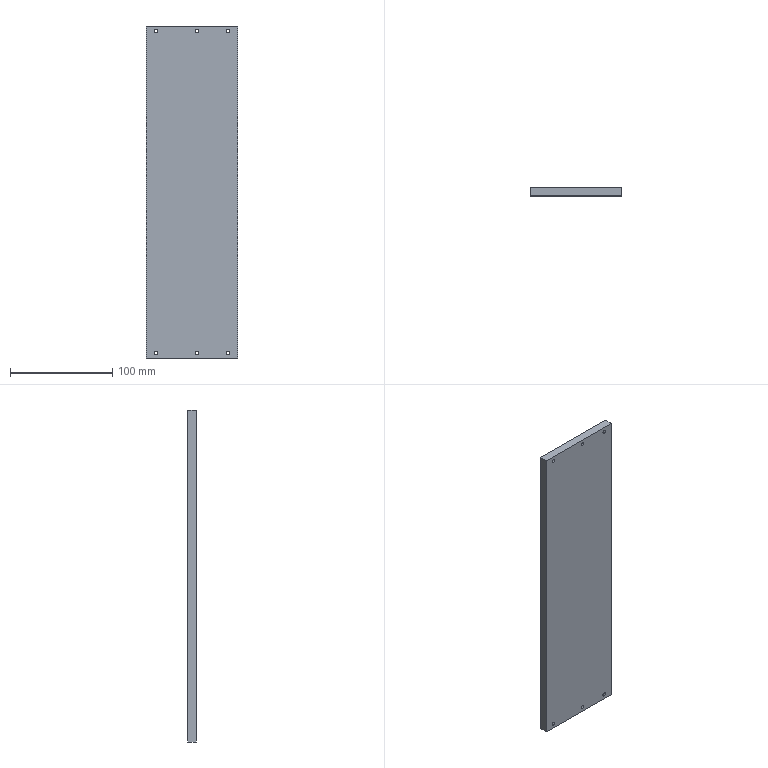Component | SolidWorks | Q1-A12-S21-Q4-12A-1 | 1 solid | 36 faces | box 90 x 8 x 325 mm | volume 233130 mm3 | cylinder 24 | plane 12 | commonest cylinder face diameters 6.5 x12 3.4 x12 | material White Plastic Steel POM
build123d program:
from build123d import *

# Parameters (mm, degrees)
SKETCH1_W                                            = 325
SKETCH1_H                                            = 90
BOSS_EXTRUDE1_DEPTH                                  = 8
M3_SOCKET_HEAD_CAP_SCREW_CYLINDRICAL_COU_D           = 3.4
M3_SOCKET_HEAD_CAP_SCREW_CYLINDRICAL_COU_CBORE_D     = 6.5
M3_SOCKET_HEAD_CAP_SCREW_CYLINDRICAL_COU_CBORE_DEPTH = 3


with BuildPart() as part:
    # Sketch1 → Boss-Extrude1 (new body)
    with BuildSketch(Plane(origin=(0, 0, 0), x_dir=(1, 0, 0), z_dir=(0, 1, 0))):
        Rectangle(SKETCH1_W, SKETCH1_H)
    extrude(amount=BOSS_EXTRUDE1_DEPTH)

    # M3 Socket Head Cap Screw Cylindrical Cou (through all)
    with Locations(Plane(origin=(0, 8, 0), x_dir=(1, 0, 0), z_dir=(0, 1, 0))):
        with Locations((157.5, 35), (157.5, 5), (157.5, -35), (-157.5, 35), (-157.5, 5), (-157.5, -35)):
            CounterBoreHole(M3_SOCKET_HEAD_CAP_SCREW_CYLINDRICAL_COU_D / 2, M3_SOCKET_HEAD_CAP_SCREW_CYLINDRICAL_COU_CBORE_D / 2, M3_SOCKET_HEAD_CAP_SCREW_CYLINDRICAL_COU_CBORE_DEPTH)


solid = part.part

# Placed as in the assembly
solid = solid.moved(Location((263.5, 180, 0), (0, -90, 0)))
STEP:
#1=COLOUR_RGB('',0.7922,0.8196,0.9333);
#2=FILL_AREA_STYLE_COLOUR('',#1);
#3=FILL_AREA_STYLE('',(#2));
#4=SURFACE_STYLE_FILL_AREA(#3);
#5=SURFACE_SIDE_STYLE('',(#4));
#6=SURFACE_STYLE_USAGE(.BOTH.,#5);
#7=PRESENTATION_STYLE_ASSIGNMENT((#6));
#8=CARTESIAN_POINT('',(11.88,7.283,6.201));
#9=VERTEX_POINT('',#8);
#10=CARTESIAN_POINT('',(11.624,7.283,6.201));
#11=VERTEX_POINT('',#10);
#12=CARTESIAN_POINT('',(11.752,7.283,6.201));
#13=DIRECTION('',(-0.,1.,0.));
#14=DIRECTION('',(-1.,0.,0.));
#15=AXIS2_PLACEMENT_3D('',#12,#13,#14);
#16=CIRCLE('',#15,0.128);
#17=EDGE_CURVE('',#9,#11,#16,.T.);
#18=ORIENTED_EDGE('',*,*,#17,.F.);
#19=CARTESIAN_POINT('',(11.88,7.402,6.201));
#20=VERTEX_POINT('',#19);
#21=CARTESIAN_POINT('',(11.88,7.402,6.201));
#22=DIRECTION('',(-0.,1.,0.));
#23=VECTOR('',#22,39.37);
#24=LINE('',#21,#23);
#25=EDGE_CURVE('',#9,#20,#24,.T.);
#26=ORIENTED_EDGE('',*,*,#25,.T.);
#27=CARTESIAN_POINT('',(11.624,7.402,6.201));
#28=VERTEX_POINT('',#27);
#29=CARTESIAN_POINT('',(11.752,7.402,6.201));
#30=DIRECTION('',(-0.,1.,0.));
#31=DIRECTION('',(-1.,0.,0.));
#32=AXIS2_PLACEMENT_3D('',#29,#30,#31);
#33=CIRCLE('',#32,0.128);
#34=EDGE_CURVE('',#20,#28,#33,.T.);
#35=ORIENTED_EDGE('',*,*,#34,.T.);
#36=CARTESIAN_POINT('',(11.624,7.402,6.201));
#37=DIRECTION('',(-0.,1.,0.));
#38=VECTOR('',#37,39.37);
#39=LINE('',#36,#38);
#40=EDGE_CURVE('',#11,#28,#39,.T.);
#41=ORIENTED_EDGE('',*,*,#40,.F.);
#42=EDGE_LOOP('',(#18,#26,#35,#41));
#43=FACE_OUTER_BOUND('',#42,.T.);
#44=CARTESIAN_POINT('',(11.752,7.402,6.201));
#45=DIRECTION('',(-0.,1.,0.));
#46=DIRECTION('',(-1.,0.,0.));
#47=AXIS2_PLACEMENT_3D('',#44,#45,#46);
#48=CYLINDRICAL_SURFACE('',#47,0.128);
#49=ADVANCED_FACE('',(#43),#48,.F.);
#50=CARTESIAN_POINT('',(11.819,7.087,6.201));
#51=VERTEX_POINT('',#50);
#52=CARTESIAN_POINT('',(11.685,7.087,6.201));
#53=VERTEX_POINT('',#52);
#54=CARTESIAN_POINT('',(11.752,7.087,6.201));
#55=DIRECTION('',(-0.,1.,0.));
#56=DIRECTION('',(-1.,0.,0.));
#57=AXIS2_PLACEMENT_3D('',#54,#55,#56);
#58=CIRCLE('',#57,0.06693);
#59=EDGE_CURVE('',#51,#53,#58,.T.);
#60=ORIENTED_EDGE('',*,*,#59,.F.);
#61=CARTESIAN_POINT('',(11.819,7.283,6.201));
#62=VERTEX_POINT('',#61);
#63=CARTESIAN_POINT('',(11.819,7.402,6.201));
#64=DIRECTION('',(-0.,1.,0.));
#65=VECTOR('',#64,39.37);
#66=LINE('',#63,#65);
#67=EDGE_CURVE('',#51,#62,#66,.T.);
#68=ORIENTED_EDGE('',*,*,#67,.T.);
#69=CARTESIAN_POINT('',(11.685,7.283,6.201));
#70=VERTEX_POINT('',#69);
#71=CARTESIAN_POINT('',(11.752,7.283,6.201));
#72=DIRECTION('',(-0.,1.,0.));
#73=DIRECTION('',(-1.,0.,0.));
#74=AXIS2_PLACEMENT_3D('',#71,#72,#73);
#75=CIRCLE('',#74,0.06693);
#76=EDGE_CURVE('',#62,#70,#75,.T.);
#77=ORIENTED_EDGE('',*,*,#76,.T.);
#78=CARTESIAN_POINT('',(11.685,7.402,6.201));
#79=DIRECTION('',(-0.,1.,0.));
#80=VECTOR('',#79,39.37);
#81=LINE('',#78,#80);
#82=EDGE_CURVE('',#53,#70,#81,.T.);
#83=ORIENTED_EDGE('',*,*,#82,.F.);
#84=EDGE_LOOP('',(#60,#68,#77,#83));
#85=FACE_OUTER_BOUND('',#84,.T.);
#86=CARTESIAN_POINT('',(11.752,7.402,6.201));
#87=DIRECTION('',(-0.,1.,0.));
#88=DIRECTION('',(-1.,0.,0.));
#89=AXIS2_PLACEMENT_3D('',#86,#87,#88);
#90=CYLINDRICAL_SURFACE('',#89,0.06693);
#91=ADVANCED_FACE('',(#85),#90,.F.);
#92=CARTESIAN_POINT('',(10.699,7.283,6.201));
#93=VERTEX_POINT('',#92);
#94=CARTESIAN_POINT('',(10.443,7.283,6.201));
#95=VERTEX_POINT('',#94);
#96=CARTESIAN_POINT('',(10.571,7.283,6.201));
#97=DIRECTION('',(-0.,1.,0.));
#98=DIRECTION('',(-1.,0.,0.));
#99=AXIS2_PLACEMENT_3D('',#96,#97,#98);
#100=CIRCLE('',#99,0.128);
#101=EDGE_CURVE('',#93,#95,#100,.T.);
#102=ORIENTED_EDGE('',*,*,#101,.F.);
#103=CARTESIAN_POINT('',(10.699,7.402,6.201));
#104=VERTEX_POINT('',#103);
#105=CARTESIAN_POINT('',(10.699,7.402,6.201));
#106=DIRECTION('',(-0.,1.,0.));
#107=VECTOR('',#106,39.37);
#108=LINE('',#105,#107);
#109=EDGE_CURVE('',#93,#104,#108,.T.);
#110=ORIENTED_EDGE('',*,*,#109,.T.);
#111=CARTESIAN_POINT('',(10.443,7.402,6.201));
#112=VERTEX_POINT('',#111);
#113=CARTESIAN_POINT('',(10.571,7.402,6.201));
#114=DIRECTION('',(-0.,1.,0.));
#115=DIRECTION('',(-1.,0.,0.));
#116=AXIS2_PLACEMENT_3D('',#113,#114,#115);
#117=CIRCLE('',#116,0.128);
#118=EDGE_CURVE('',#104,#112,#117,.T.);
#119=ORIENTED_EDGE('',*,*,#118,.T.);
#120=CARTESIAN_POINT('',(10.443,7.402,6.201));
#121=DIRECTION('',(-0.,1.,0.));
#122=VECTOR('',#121,39.37);
#123=LINE('',#120,#122);
#124=EDGE_CURVE('',#95,#112,#123,.T.);
#125=ORIENTED_EDGE('',*,*,#124,.F.);
#126=EDGE_LOOP('',(#102,#110,#119,#125));
#127=FACE_OUTER_BOUND('',#126,.T.);
#128=CARTESIAN_POINT('',(10.571,7.402,6.201));
#129=DIRECTION('',(-0.,1.,0.));
#130=DIRECTION('',(-1.,0.,0.));
#131=AXIS2_PLACEMENT_3D('',#128,#129,#130);
#132=CYLINDRICAL_SURFACE('',#131,0.128);
#133=ADVANCED_FACE('',(#127),#132,.F.);
#134=CARTESIAN_POINT('',(10.638,7.087,6.201));
#135=VERTEX_POINT('',#134);
#136=CARTESIAN_POINT('',(10.504,7.087,6.201));
#137=VERTEX_POINT('',#136);
#138=CARTESIAN_POINT('',(10.571,7.087,6.201));
#139=DIRECTION('',(-0.,1.,0.));
#140=DIRECTION('',(-1.,0.,0.));
#141=AXIS2_PLACEMENT_3D('',#138,#139,#140);
#142=CIRCLE('',#141,0.06693);
#143=EDGE_CURVE('',#135,#137,#142,.T.);
#144=ORIENTED_EDGE('',*,*,#143,.F.);
#145=CARTESIAN_POINT('',(10.638,7.283,6.201));
#146=VERTEX_POINT('',#145);
#147=CARTESIAN_POINT('',(10.638,7.402,6.201));
#148=DIRECTION('',(-0.,1.,0.));
#149=VECTOR('',#148,39.37);
#150=LINE('',#147,#149);
#151=EDGE_CURVE('',#135,#146,#150,.T.);
#152=ORIENTED_EDGE('',*,*,#151,.T.);
#153=CARTESIAN_POINT('',(10.504,7.283,6.201));
#154=VERTEX_POINT('',#153);
#155=CARTESIAN_POINT('',(10.571,7.283,6.201));
#156=DIRECTION('',(-0.,1.,0.));
#157=DIRECTION('',(-1.,0.,0.));
#158=AXIS2_PLACEMENT_3D('',#155,#156,#157);
#159=CIRCLE('',#158,0.06693);
#160=EDGE_CURVE('',#146,#154,#159,.T.);
#161=ORIENTED_EDGE('',*,*,#160,.T.);
#162=CARTESIAN_POINT('',(10.504,7.402,6.201));
#163=DIRECTION('',(-0.,1.,0.));
#164=VECTOR('',#163,39.37);
#165=LINE('',#162,#164);
#166=EDGE_CURVE('',#137,#154,#165,.T.);
#167=ORIENTED_EDGE('',*,*,#166,.F.);
#168=EDGE_LOOP('',(#144,#152,#161,#167));
#169=FACE_OUTER_BOUND('',#168,.T.);
#170=CARTESIAN_POINT('',(10.571,7.402,6.201));
#171=DIRECTION('',(-0.,1.,0.));
#172=DIRECTION('',(-1.,0.,0.));
#173=AXIS2_PLACEMENT_3D('',#170,#171,#172);
#174=CYLINDRICAL_SURFACE('',#173,0.06693);
#175=ADVANCED_FACE('',(#169),#174,.F.);
#176=CARTESIAN_POINT('',(9.124,7.283,6.201));
#177=VERTEX_POINT('',#176);
#178=CARTESIAN_POINT('',(8.868,7.283,6.201));
#179=VERTEX_POINT('',#178);
#180=CARTESIAN_POINT('',(8.996,7.283,6.201));
#181=DIRECTION('',(-0.,1.,0.));
#182=DIRECTION('',(-1.,0.,0.));
#183=AXIS2_PLACEMENT_3D('',#180,#181,#182);
#184=CIRCLE('',#183,0.128);
#185=EDGE_CURVE('',#177,#179,#184,.T.);
#186=ORIENTED_EDGE('',*,*,#185,.F.);
#187=CARTESIAN_POINT('',(9.124,7.402,6.201));
#188=VERTEX_POINT('',#187);
#189=CARTESIAN_POINT('',(9.124,7.402,6.201));
#190=DIRECTION('',(-0.,1.,0.));
#191=VECTOR('',#190,39.37);
#192=LINE('',#189,#191);
#193=EDGE_CURVE('',#177,#188,#192,.T.);
#194=ORIENTED_EDGE('',*,*,#193,.T.);
#195=CARTESIAN_POINT('',(8.868,7.402,6.201));
#196=VERTEX_POINT('',#195);
#197=CARTESIAN_POINT('',(8.996,7.402,6.201));
#198=DIRECTION('',(-0.,1.,0.));
#199=DIRECTION('',(-1.,0.,0.));
#200=AXIS2_PLACEMENT_3D('',#197,#198,#199);
#201=CIRCLE('',#200,0.128);
#202=EDGE_CURVE('',#188,#196,#201,.T.);
#203=ORIENTED_EDGE('',*,*,#202,.T.);
#204=CARTESIAN_POINT('',(8.868,7.402,6.201));
#205=DIRECTION('',(-0.,1.,0.));
#206=VECTOR('',#205,39.37);
#207=LINE('',#204,#206);
#208=EDGE_CURVE('',#179,#196,#207,.T.);
#209=ORIENTED_EDGE('',*,*,#208,.F.);
#210=EDGE_LOOP('',(#186,#194,#203,#209));
#211=FACE_OUTER_BOUND('',#210,.T.);
#212=CARTESIAN_POINT('',(8.996,7.402,6.201));
#213=DIRECTION('',(-0.,1.,0.));
#214=DIRECTION('',(-1.,0.,0.));
#215=AXIS2_PLACEMENT_3D('',#212,#213,#214);
#216=CYLINDRICAL_SURFACE('',#215,0.128);
#217=ADVANCED_FACE('',(#211),#216,.F.);
#218=CARTESIAN_POINT('',(9.063,7.087,6.201));
#219=VERTEX_POINT('',#218);
#220=CARTESIAN_POINT('',(8.929,7.087,6.201));
#221=VERTEX_POINT('',#220);
#222=CARTESIAN_POINT('',(8.996,7.087,6.201));
#223=DIRECTION('',(-0.,1.,0.));
#224=DIRECTION('',(-1.,0.,0.));
#225=AXIS2_PLACEMENT_3D('',#222,#223,#224);
#226=CIRCLE('',#225,0.06693);
#227=EDGE_CURVE('',#219,#221,#226,.T.);
#228=ORIENTED_EDGE('',*,*,#227,.F.);
#229=CARTESIAN_POINT('',(9.063,7.283,6.201));
#230=VERTEX_POINT('',#229);
#231=CARTESIAN_POINT('',(9.063,7.402,6.201));
#232=DIRECTION('',(-0.,1.,0.));
#233=VECTOR('',#232,39.37);
#234=LINE('',#231,#233);
#235=EDGE_CURVE('',#219,#230,#234,.T.);
#236=ORIENTED_EDGE('',*,*,#235,.T.);
#237=CARTESIAN_POINT('',(8.929,7.283,6.201));
#238=VERTEX_POINT('',#237);
#239=CARTESIAN_POINT('',(8.996,7.283,6.201));
#240=DIRECTION('',(-0.,1.,0.));
#241=DIRECTION('',(-1.,0.,0.));
#242=AXIS2_PLACEMENT_3D('',#239,#240,#241);
#243=CIRCLE('',#242,0.06693);
#244=EDGE_CURVE('',#230,#238,#243,.T.);
#245=ORIENTED_EDGE('',*,*,#244,.T.);
#246=CARTESIAN_POINT('',(8.929,7.402,6.201));
#247=DIRECTION('',(-0.,1.,0.));
#248=VECTOR('',#247,39.37);
#249=LINE('',#246,#248);
#250=EDGE_CURVE('',#221,#238,#249,.T.);
#251=ORIENTED_EDGE('',*,*,#250,.F.);
#252=EDGE_LOOP('',(#228,#236,#245,#251));
#253=FACE_OUTER_BOUND('',#252,.T.);
#254=CARTESIAN_POINT('',(8.996,7.402,6.201));
#255=DIRECTION('',(-0.,1.,0.));
#256=DIRECTION('',(-1.,0.,0.));
#257=AXIS2_PLACEMENT_3D('',#254,#255,#256);
#258=CYLINDRICAL_SURFACE('',#257,0.06693);
#259=ADVANCED_FACE('',(#253),#258,.F.);
#260=CARTESIAN_POINT('',(11.88,7.283,-6.201));
#261=VERTEX_POINT('',#260);
#262=CARTESIAN_POINT('',(11.624,7.283,-6.201));
#263=VERTEX_POINT('',#262);
#264=CARTESIAN_POINT('',(11.752,7.283,-6.201));
#265=DIRECTION('',(-0.,1.,0.));
#266=DIRECTION('',(-1.,0.,0.));
#267=AXIS2_PLACEMENT_3D('',#264,#265,#266);
#268=CIRCLE('',#267,0.128);
#269=EDGE_CURVE('',#261,#263,#268,.T.);
#270=ORIENTED_EDGE('',*,*,#269,.F.);
#271=CARTESIAN_POINT('',(11.88,7.402,-6.201));
#272=VERTEX_POINT('',#271);
#273=CARTESIAN_POINT('',(11.88,7.402,-6.201));
#274=DIRECTION('',(-0.,1.,0.));
#275=VECTOR('',#274,39.37);
#276=LINE('',#273,#275);
#277=EDGE_CURVE('',#261,#272,#276,.T.);
#278=ORIENTED_EDGE('',*,*,#277,.T.);
#279=CARTESIAN_POINT('',(11.624,7.402,-6.201));
#280=VERTEX_POINT('',#279);
#281=CARTESIAN_POINT('',(11.752,7.402,-6.201));
#282=DIRECTION('',(-0.,1.,0.));
#283=DIRECTION('',(-1.,0.,0.));
#284=AXIS2_PLACEMENT_3D('',#281,#282,#283);
#285=CIRCLE('',#284,0.128);
#286=EDGE_CURVE('',#272,#280,#285,.T.);
#287=ORIENTED_EDGE('',*,*,#286,.T.);
#288=CARTESIAN_POINT('',(11.624,7.402,-6.201));
#289=DIRECTION('',(-0.,1.,0.));
#290=VECTOR('',#289,39.37);
#291=LINE('',#288,#290);
#292=EDGE_CURVE('',#263,#280,#291,.T.);
#293=ORIENTED_EDGE('',*,*,#292,.F.);
#294=EDGE_LOOP('',(#270,#278,#287,#293));
#295=FACE_OUTER_BOUND('',#294,.T.);
#296=CARTESIAN_POINT('',(11.752,7.402,-6.201));
#297=DIRECTION('',(-0.,1.,0.));
#298=DIRECTION('',(-1.,0.,0.));
#299=AXIS2_PLACEMENT_3D('',#296,#297,#298);
#300=CYLINDRICAL_SURFACE('',#299,0.128);
#301=ADVANCED_FACE('',(#295),#300,.F.);
#302=CARTESIAN_POINT('',(11.819,7.087,-6.201));
#303=VERTEX_POINT('',#302);
#304=CARTESIAN_POINT('',(11.685,7.087,-6.201));
#305=VERTEX_POINT('',#304);
#306=CARTESIAN_POINT('',(11.752,7.087,-6.201));
#307=DIRECTION('',(-0.,1.,0.));
#308=DIRECTION('',(-1.,0.,0.));
#309=AXIS2_PLACEMENT_3D('',#306,#307,#308);
#310=CIRCLE('',#309,0.06693);
#311=EDGE_CURVE('',#303,#305,#310,.T.);
#312=ORIENTED_EDGE('',*,*,#311,.F.);
#313=CARTESIAN_POINT('',(11.819,7.283,-6.201));
#314=VERTEX_POINT('',#313);
#315=CARTESIAN_POINT('',(11.819,7.402,-6.201));
#316=DIRECTION('',(-0.,1.,0.));
#317=VECTOR('',#316,39.37);
#318=LINE('',#315,#317);
#319=EDGE_CURVE('',#303,#314,#318,.T.);
#320=ORIENTED_EDGE('',*,*,#319,.T.);
#321=CARTESIAN_POINT('',(11.685,7.283,-6.201));
#322=VERTEX_POINT('',#321);
#323=CARTESIAN_POINT('',(11.752,7.283,-6.201));
#324=DIRECTION('',(-0.,1.,0.));
#325=DIRECTION('',(-1.,0.,0.));
#326=AXIS2_PLACEMENT_3D('',#323,#324,#325);
#327=CIRCLE('',#326,0.06693);
#328=EDGE_CURVE('',#314,#322,#327,.T.);
#329=ORIENTED_EDGE('',*,*,#328,.T.);
#330=CARTESIAN_POINT('',(11.685,7.402,-6.201));
#331=DIRECTION('',(-0.,1.,0.));
#332=VECTOR('',#331,39.37);
#333=LINE('',#330,#332);
#334=EDGE_CURVE('',#305,#322,#333,.T.);
#335=ORIENTED_EDGE('',*,*,#334,.F.);
#336=EDGE_LOOP('',(#312,#320,#329,#335));
#337=FACE_OUTER_BOUND('',#336,.T.);
#338=CARTESIAN_POINT('',(11.752,7.402,-6.201));
#339=DIRECTION('',(-0.,1.,0.));
#340=DIRECTION('',(-1.,0.,0.));
#341=AXIS2_PLACEMENT_3D('',#338,#339,#340);
#342=CYLINDRICAL_SURFACE('',#341,0.06693);
#343=ADVANCED_FACE('',(#337),#342,.F.);
#344=CARTESIAN_POINT('',(10.699,7.283,-6.201));
#345=VERTEX_POINT('',#344);
#346=CARTESIAN_POINT('',(10.443,7.283,-6.201));
#347=VERTEX_POINT('',#346);
#348=CARTESIAN_POINT('',(10.571,7.283,-6.201));
#349=DIRECTION('',(-0.,1.,0.));
#350=DIRECTION('',(-1.,0.,0.));
#351=AXIS2_PLACEMENT_3D('',#348,#349,#350);
#352=CIRCLE('',#351,0.128);
#353=EDGE_CURVE('',#345,#347,#352,.T.);
#354=ORIENTED_EDGE('',*,*,#353,.F.);
#355=CARTESIAN_POINT('',(10.699,7.402,-6.201));
#356=VERTEX_POINT('',#355);
#357=CARTESIAN_POINT('',(10.699,7.402,-6.201));
#358=DIRECTION('',(-0.,1.,0.));
#359=VECTOR('',#358,39.37);
#360=LINE('',#357,#359);
#361=EDGE_CURVE('',#345,#356,#360,.T.);
#362=ORIENTED_EDGE('',*,*,#361,.T.);
#363=CARTESIAN_POINT('',(10.443,7.402,-6.201));
#364=VERTEX_POINT('',#363);
#365=CARTESIAN_POINT('',(10.571,7.402,-6.201));
#366=DIRECTION('',(-0.,1.,0.));
#367=DIRECTION('',(-1.,0.,0.));
#368=AXIS2_PLACEMENT_3D('',#365,#366,#367);
#369=CIRCLE('',#368,0.128);
#370=EDGE_CURVE('',#356,#364,#369,.T.);
#371=ORIENTED_EDGE('',*,*,#370,.T.);
#372=CARTESIAN_POINT('',(10.443,7.402,-6.201));
#373=DIRECTION('',(-0.,1.,0.));
#374=VECTOR('',#373,39.37);
#375=LINE('',#372,#374);
#376=EDGE_CURVE('',#347,#364,#375,.T.);
#377=ORIENTED_EDGE('',*,*,#376,.F.);
#378=EDGE_LOOP('',(#354,#362,#371,#377));
#379=FACE_OUTER_BOUND('',#378,.T.);
#380=CARTESIAN_POINT('',(10.571,7.402,-6.201));
#381=DIRECTION('',(-0.,1.,0.));
#382=DIRECTION('',(-1.,0.,0.));
#383=AXIS2_PLACEMENT_3D('',#380,#381,#382);
#384=CYLINDRICAL_SURFACE('',#383,0.128);
#385=ADVANCED_FACE('',(#379),#384,.F.);
#386=CARTESIAN_POINT('',(10.638,7.087,-6.201));
#387=VERTEX_POINT('',#386);
#388=CARTESIAN_POINT('',(10.504,7.087,-6.201));
#389=VERTEX_POINT('',#388);
#390=CARTESIAN_POINT('',(10.571,7.087,-6.201));
#391=DIRECTION('',(-0.,1.,0.));
#392=DIRECTION('',(-1.,0.,0.));
#393=AXIS2_PLACEMENT_3D('',#390,#391,#392);
#394=CIRCLE('',#393,0.06693);
#395=EDGE_CURVE('',#387,#389,#394,.T.);
#396=ORIENTED_EDGE('',*,*,#395,.F.);
#397=CARTESIAN_POINT('',(10.638,7.283,-6.201));
#398=VERTEX_POINT('',#397);
#399=CARTESIAN_POINT('',(10.638,7.402,-6.201));
#400=DIRECTION('',(-0.,1.,0.));
#401=VECTOR('',#400,39.37);
#402=LINE('',#399,#401);
#403=EDGE_CURVE('',#387,#398,#402,.T.);
#404=ORIENTED_EDGE('',*,*,#403,.T.);
#405=CARTESIAN_POINT('',(10.504,7.283,-6.201));
#406=VERTEX_POINT('',#405);
#407=CARTESIAN_POINT('',(10.571,7.283,-6.201));
#408=DIRECTION('',(-0.,1.,0.));
#409=DIRECTION('',(-1.,0.,0.));
#410=AXIS2_PLACEMENT_3D('',#407,#408,#409);
#411=CIRCLE('',#410,0.06693);
#412=EDGE_CURVE('',#398,#406,#411,.T.);
#413=ORIENTED_EDGE('',*,*,#412,.T.);
#414=CARTESIAN_POINT('',(10.504,7.402,-6.201));
#415=DIRECTION('',(-0.,1.,0.));
#416=VECTOR('',#415,39.37);
#417=LINE('',#414,#416);
#418=EDGE_CURVE('',#389,#406,#417,.T.);
#419=ORIENTED_EDGE('',*,*,#418,.F.);
#420=EDGE_LOOP('',(#396,#404,#413,#419));
#421=FACE_OUTER_BOUND('',#420,.T.);
#422=CARTESIAN_POINT('',(10.571,7.402,-6.201));
#423=DIRECTION('',(-0.,1.,0.));
#424=DIRECTION('',(-1.,0.,0.));
#425=AXIS2_PLACEMENT_3D('',#422,#423,#424);
#426=CYLINDRICAL_SURFACE('',#425,0.06693);
#427=ADVANCED_FACE('',(#421),#426,.F.);
#428=CARTESIAN_POINT('',(9.124,7.283,-6.201));
#429=VERTEX_POINT('',#428);
#430=CARTESIAN_POINT('',(8.868,7.283,-6.201));
#431=VERTEX_POINT('',#430);
#432=CARTESIAN_POINT('',(8.996,7.283,-6.201));
#433=DIRECTION('',(-0.,1.,0.));
#434=DIRECTION('',(-1.,0.,0.));
#435=AXIS2_PLACEMENT_3D('',#432,#433,#434);
#436=CIRCLE('',#435,0.128);
#437=EDGE_CURVE('',#429,#431,#436,.T.);
#438=ORIENTED_EDGE('',*,*,#437,.F.);
#439=CARTESIAN_POINT('',(9.124,7.402,-6.201));
#440=VERTEX_POINT('',#439);
#441=CARTESIAN_POINT('',(9.124,7.402,-6.201));
#442=DIRECTION('',(-0.,1.,0.));
#443=VECTOR('',#442,39.37);
#444=LINE('',#441,#443);
#445=EDGE_CURVE('',#429,#440,#444,.T.);
#446=ORIENTED_EDGE('',*,*,#445,.T.);
#447=CARTESIAN_POINT('',(8.868,7.402,-6.201));
#448=VERTEX_POINT('',#447);
#449=CARTESIAN_POINT('',(8.996,7.402,-6.201));
#450=DIRECTION('',(-0.,1.,0.));
#451=DIRECTION('',(-1.,0.,0.));
#452=AXIS2_PLACEMENT_3D('',#449,#450,#451);
#453=CIRCLE('',#452,0.128);
#454=EDGE_CURVE('',#440,#448,#453,.T.);
#455=ORIENTED_EDGE('',*,*,#454,.T.);
#456=CARTESIAN_POINT('',(8.868,7.402,-6.201));
#457=DIRECTION('',(-0.,1.,0.));
#458=VECTOR('',#457,39.37);
#459=LINE('',#456,#458);
#460=EDGE_CURVE('',#431,#448,#459,.T.);
#461=ORIENTED_EDGE('',*,*,#460,.F.);
#462=EDGE_LOOP('',(#438,#446,#455,#461));
#463=FACE_OUTER_BOUND('',#462,.T.);
#464=CARTESIAN_POINT('',(8.996,7.402,-6.201));
#465=DIRECTION('',(-0.,1.,0.));
#466=DIRECTION('',(-1.,0.,0.));
#467=AXIS2_PLACEMENT_3D('',#464,#465,#466);
#468=CYLINDRICAL_SURFACE('',#467,0.128);
#469=ADVANCED_FACE('',(#463),#468,.F.);
#470=CARTESIAN_POINT('',(9.063,7.087,-6.201));
#471=VERTEX_POINT('',#470);
#472=CARTESIAN_POINT('',(8.929,7.087,-6.201));
#473=VERTEX_POINT('',#472);
#474=CARTESIAN_POINT('',(8.996,7.087,-6.201));
#475=DIRECTION('',(-0.,1.,0.));
#476=DIRECTION('',(-1.,0.,0.));
#477=AXIS2_PLACEMENT_3D('',#474,#475,#476);
#478=CIRCLE('',#477,0.06693);
#479=EDGE_CURVE('',#471,#473,#478,.T.);
#480=ORIENTED_EDGE('',*,*,#479,.F.);
#481=CARTESIAN_POINT('',(9.063,7.283,-6.201));
#482=VERTEX_POINT('',#481);
#483=CARTESIAN_POINT('',(9.063,7.402,-6.201));
#484=DIRECTION('',(-0.,1.,0.));
#485=VECTOR('',#484,39.37);
#486=LINE('',#483,#485);
#487=EDGE_CURVE('',#471,#482,#486,.T.);
#488=ORIENTED_EDGE('',*,*,#487,.T.);
#489=CARTESIAN_POINT('',(8.929,7.283,-6.201));
#490=VERTEX_POINT('',#489);
#491=CARTESIAN_POINT('',(8.996,7.283,-6.201));
#492=DIRECTION('',(-0.,1.,0.));
#493=DIRECTION('',(-1.,0.,0.));
#494=AXIS2_PLACEMENT_3D('',#491,#492,#493);
#495=CIRCLE('',#494,0.06693);
#496=EDGE_CURVE('',#482,#490,#495,.T.);
#497=ORIENTED_EDGE('',*,*,#496,.T.);
#498=CARTESIAN_POINT('',(8.929,7.402,-6.201));
#499=DIRECTION('',(-0.,1.,0.));
#500=VECTOR('',#499,39.37);
#501=LINE('',#498,#500);
#502=EDGE_CURVE('',#473,#490,#501,.T.);
#503=ORIENTED_EDGE('',*,*,#502,.F.);
#504=EDGE_LOOP('',(#480,#488,#497,#503));
#505=FACE_OUTER_BOUND('',#504,.T.);
#506=CARTESIAN_POINT('',(8.996,7.402,-6.201));
#507=DIRECTION('',(-0.,1.,0.));
#508=DIRECTION('',(-1.,0.,0.));
#509=AXIS2_PLACEMENT_3D('',#506,#507,#508);
#510=CYLINDRICAL_SURFACE('',#509,0.06693);
#511=ADVANCED_FACE('',(#505),#510,.F.);
#512=CARTESIAN_POINT('',(8.602,7.087,6.398));
#513=VERTEX_POINT('',#512);
#514=CARTESIAN_POINT('',(12.146,7.087,6.398));
#515=VERTEX_POINT('',#514);
#516=CARTESIAN_POINT('',(8.602,7.087,6.398));
#517=DIRECTION('',(1.,-0.,0.));
#518=VECTOR('',#517,39.37);
#519=LINE('',#516,#518);
#520=EDGE_CURVE('',#513,#515,#519,.T.);
#521=ORIENTED_EDGE('',*,*,#520,.T.);
#522=CARTESIAN_POINT('',(12.146,7.402,6.398));
#523=VERTEX_POINT('',#522);
#524=CARTESIAN_POINT('',(12.146,7.402,6.398));
#525=DIRECTION('',(0.,-1.,-0.));
#526=VECTOR('',#525,39.37);
#527=LINE('',#524,#526);
#528=EDGE_CURVE('',#523,#515,#527,.T.);
#529=ORIENTED_EDGE('',*,*,#528,.F.);
#530=CARTESIAN_POINT('',(8.602,7.402,6.398));
#531=VERTEX_POINT('',#530);
#532=CARTESIAN_POINT('',(8.602,7.402,6.398));
#533=DIRECTION('',(1.,-0.,0.));
#534=VECTOR('',#533,39.37);
#535=LINE('',#532,#534);
#536=EDGE_CURVE('',#531,#523,#535,.T.);
#537=ORIENTED_EDGE('',*,*,#536,.F.);
#538=CARTESIAN_POINT('',(8.602,7.402,6.398));
#539=DIRECTION('',(0.,-1.,-0.));
#540=VECTOR('',#539,39.37);
#541=LINE('',#538,#540);
#542=EDGE_CURVE('',#531,#513,#541,.T.);
#543=ORIENTED_EDGE('',*,*,#542,.T.);
#544=EDGE_LOOP('',(#521,#529,#537,#543));
#545=FACE_OUTER_BOUND('',#544,.T.);
#546=CARTESIAN_POINT('',(8.602,7.402,6.398));
#547=DIRECTION('',(0.,0.,-1.));
#548=DIRECTION('',(-1.,0.,-0.));
#549=AXIS2_PLACEMENT_3D('',#546,#547,#548);
#550=PLANE('',#549);
#551=ADVANCED_FACE('',(#545),#550,.F.);
#552=CARTESIAN_POINT('',(12.146,7.087,-6.398));
#553=VERTEX_POINT('',#552);
#554=CARTESIAN_POINT('',(12.146,7.087,-6.398));
#555=DIRECTION('',(0.,0.,-1.));
#556=VECTOR('',#555,39.37);
#557=LINE('',#554,#556);
#558=EDGE_CURVE('',#515,#553,#557,.T.);
#559=ORIENTED_EDGE('',*,*,#558,.T.);
#560=CARTESIAN_POINT('',(12.146,7.402,-6.398));
#561=VERTEX_POINT('',#560);
#562=CARTESIAN_POINT('',(12.146,7.402,-6.398));
#563=DIRECTION('',(0.,-1.,-0.));
#564=VECTOR('',#563,39.37);
#565=LINE('',#562,#564);
#566=EDGE_CURVE('',#561,#553,#565,.T.);
#567=ORIENTED_EDGE('',*,*,#566,.F.);
#568=CARTESIAN_POINT('',(12.146,7.402,-6.398));
#569=DIRECTION('',(0.,0.,-1.));
#570=VECTOR('',#569,39.37);
#571=LINE('',#568,#570);
#572=EDGE_CURVE('',#523,#561,#571,.T.);
#573=ORIENTED_EDGE('',*,*,#572,.F.);
#574=ORIENTED_EDGE('',*,*,#528,.T.);
#575=EDGE_LOOP('',(#559,#567,#573,#574));
#576=FACE_OUTER_BOUND('',#575,.T.);
#577=CARTESIAN_POINT('',(12.146,7.402,-6.398));
#578=DIRECTION('',(-1.,0.,0.));
#579=DIRECTION('',(0.,-0.,1.));
#580=AXIS2_PLACEMENT_3D('',#577,#578,#579);
#581=PLANE('',#580);
#582=ADVANCED_FACE('',(#576),#581,.F.);
#583=CARTESIAN_POINT('',(8.602,7.087,-6.398));
#584=VERTEX_POINT('',#583);
#585=CARTESIAN_POINT('',(8.602,7.087,-6.398));
#586=DIRECTION('',(-1.,0.,-0.));
#587=VECTOR('',#586,39.37);
#588=LINE('',#585,#587);
#589=EDGE_CURVE('',#553,#584,#588,.T.);
#590=ORIENTED_EDGE('',*,*,#589,.T.);
#591=CARTESIAN_POINT('',(8.602,7.402,-6.398));
#592=VERTEX_POINT('',#591);
#593=CARTESIAN_POINT('',(8.602,7.402,-6.398));
#594=DIRECTION('',(0.,-1.,-0.));
#595=VECTOR('',#594,39.37);
#596=LINE('',#593,#595);
#597=EDGE_CURVE('',#592,#584,#596,.T.);
#598=ORIENTED_EDGE('',*,*,#597,.F.);
#599=CARTESIAN_POINT('',(8.602,7.402,-6.398));
#600=DIRECTION('',(-1.,0.,-0.));
#601=VECTOR('',#600,39.37);
#602=LINE('',#599,#601);
#603=EDGE_CURVE('',#561,#592,#602,.T.);
#604=ORIENTED_EDGE('',*,*,#603,.F.);
#605=ORIENTED_EDGE('',*,*,#566,.T.);
#606=EDGE_LOOP('',(#590,#598,#604,#605));
#607=FACE_OUTER_BOUND('',#606,.T.);
#608=CARTESIAN_POINT('',(8.602,7.402,-6.398));
#609=DIRECTION('',(-0.,-0.,1.));
#610=DIRECTION('',(1.,-0.,0.));
#611=AXIS2_PLACEMENT_3D('',#608,#609,#610);
#612=PLANE('',#611);
#613=ADVANCED_FACE('',(#607),#612,.F.);
#614=CARTESIAN_POINT('',(8.602,7.087,-6.398));
#615=DIRECTION('',(0.,-0.,1.));
#616=VECTOR('',#615,39.37);
#617=LINE('',#614,#616);
#618=EDGE_CURVE('',#584,#513,#617,.T.);
#619=ORIENTED_EDGE('',*,*,#618,.T.);
#620=ORIENTED_EDGE('',*,*,#542,.F.);
#621=CARTESIAN_POINT('',(8.602,7.402,-6.398));
#622=DIRECTION('',(0.,-0.,1.));
#623=VECTOR('',#622,39.37);
#624=LINE('',#621,#623);
#625=EDGE_CURVE('',#592,#531,#624,.T.);
#626=ORIENTED_EDGE('',*,*,#625,.F.);
#627=ORIENTED_EDGE('',*,*,#597,.T.);
#628=EDGE_LOOP('',(#619,#620,#626,#627));
#629=FACE_OUTER_BOUND('',#628,.T.);
#630=CARTESIAN_POINT('',(8.602,7.402,-6.398));
#631=DIRECTION('',(1.,-0.,-0.));
#632=DIRECTION('',(0.,0.,-1.));
#633=AXIS2_PLACEMENT_3D('',#630,#631,#632);
#634=PLANE('',#633);
#635=ADVANCED_FACE('',(#629),#634,.F.);
#636=CARTESIAN_POINT('',(11.752,7.402,6.201));
#637=DIRECTION('',(-0.,1.,0.));
#638=DIRECTION('',(-1.,0.,0.));
#639=AXIS2_PLACEMENT_3D('',#636,#637,#638);
#640=CIRCLE('',#639,0.128);
#641=EDGE_CURVE('',#28,#20,#640,.T.);
#642=ORIENTED_EDGE('',*,*,#641,.F.);
#643=ORIENTED_EDGE('',*,*,#34,.F.);
#644=EDGE_LOOP('',(#642,#643));
#645=FACE_BOUND('',#644,.T.);
#646=CARTESIAN_POINT('',(10.571,7.402,6.201));
#647=DIRECTION('',(-0.,1.,0.));
#648=DIRECTION('',(-1.,0.,0.));
#649=AXIS2_PLACEMENT_3D('',#646,#647,#648);
#650=CIRCLE('',#649,0.128);
#651=EDGE_CURVE('',#112,#104,#650,.T.);
#652=ORIENTED_EDGE('',*,*,#651,.F.);
#653=ORIENTED_EDGE('',*,*,#118,.F.);
#654=EDGE_LOOP('',(#652,#653));
#655=FACE_BOUND('',#654,.T.);
#656=CARTESIAN_POINT('',(8.996,7.402,6.201));
#657=DIRECTION('',(-0.,1.,0.));
#658=DIRECTION('',(-1.,0.,0.));
#659=AXIS2_PLACEMENT_3D('',#656,#657,#658);
#660=CIRCLE('',#659,0.128);
#661=EDGE_CURVE('',#196,#188,#660,.T.);
#662=ORIENTED_EDGE('',*,*,#661,.F.);
#663=ORIENTED_EDGE('',*,*,#202,.F.);
#664=EDGE_LOOP('',(#662,#663));
#665=FACE_BOUND('',#664,.T.);
#666=CARTESIAN_POINT('',(11.752,7.402,-6.201));
#667=DIRECTION('',(-0.,1.,0.));
#668=DIRECTION('',(-1.,0.,0.));
#669=AXIS2_PLACEMENT_3D('',#666,#667,#668);
#670=CIRCLE('',#669,0.128);
#671=EDGE_CURVE('',#280,#272,#670,.T.);
#672=ORIENTED_EDGE('',*,*,#671,.F.);
#673=ORIENTED_EDGE('',*,*,#286,.F.);
#674=EDGE_LOOP('',(#672,#673));
#675=FACE_BOUND('',#674,.T.);
#676=CARTESIAN_POINT('',(10.571,7.402,-6.201));
#677=DIRECTION('',(-0.,1.,0.));
#678=DIRECTION('',(-1.,0.,0.));
#679=AXIS2_PLACEMENT_3D('',#676,#677,#678);
#680=CIRCLE('',#679,0.128);
#681=EDGE_CURVE('',#364,#356,#680,.T.);
#682=ORIENTED_EDGE('',*,*,#681,.F.);
#683=ORIENTED_EDGE('',*,*,#370,.F.);
#684=EDGE_LOOP('',(#682,#683));
#685=FACE_BOUND('',#684,.T.);
#686=CARTESIAN_POINT('',(8.996,7.402,-6.201));
#687=DIRECTION('',(-0.,1.,0.));
#688=DIRECTION('',(-1.,0.,0.));
#689=AXIS2_PLACEMENT_3D('',#686,#687,#688);
#690=CIRCLE('',#689,0.128);
#691=EDGE_CURVE('',#448,#440,#690,.T.);
#692=ORIENTED_EDGE('',*,*,#691,.F.);
#693=ORIENTED_EDGE('',*,*,#454,.F.);
#694=EDGE_LOOP('',(#692,#693));
#695=FACE_BOUND('',#694,.T.);
#696=ORIENTED_EDGE('',*,*,#536,.T.);
#697=ORIENTED_EDGE('',*,*,#572,.T.);
#698=ORIENTED_EDGE('',*,*,#603,.T.);
#699=ORIENTED_EDGE('',*,*,#625,.T.);
#700=EDGE_LOOP('',(#696,#697,#698,#699));
#701=FACE_OUTER_BOUND('',#700,.T.);
#702=CARTESIAN_POINT('',(10.374,7.402,-0.));
#703=DIRECTION('',(-0.,-1.,-0.));
#704=DIRECTION('',(1.,-0.,0.));
#705=AXIS2_PLACEMENT_3D('',#702,#703,#704);
#706=PLANE('',#705);
#707=ADVANCED_FACE('',(#645,#655,#665,#675,#685,#695,#701),#706,.F.);
#708=CARTESIAN_POINT('',(11.752,7.087,6.201));
#709=DIRECTION('',(-0.,1.,0.));
#710=DIRECTION('',(-1.,0.,0.));
#711=AXIS2_PLACEMENT_3D('',#708,#709,#710);
#712=CIRCLE('',#711,0.06693);
#713=EDGE_CURVE('',#53,#51,#712,.T.);
#714=ORIENTED_EDGE('',*,*,#713,.T.);
#715=ORIENTED_EDGE('',*,*,#59,.T.);
#716=EDGE_LOOP('',(#714,#715));
#717=FACE_BOUND('',#716,.T.);
#718=CARTESIAN_POINT('',(10.571,7.087,6.201));
#719=DIRECTION('',(-0.,1.,0.));
#720=DIRECTION('',(-1.,0.,0.));
#721=AXIS2_PLACEMENT_3D('',#718,#719,#720);
#722=CIRCLE('',#721,0.06693);
#723=EDGE_CURVE('',#137,#135,#722,.T.);
#724=ORIENTED_EDGE('',*,*,#723,.T.);
#725=ORIENTED_EDGE('',*,*,#143,.T.);
#726=EDGE_LOOP('',(#724,#725));
#727=FACE_BOUND('',#726,.T.);
#728=CARTESIAN_POINT('',(8.996,7.087,6.201));
#729=DIRECTION('',(-0.,1.,0.));
#730=DIRECTION('',(-1.,0.,0.));
#731=AXIS2_PLACEMENT_3D('',#728,#729,#730);
#732=CIRCLE('',#731,0.06693);
#733=EDGE_CURVE('',#221,#219,#732,.T.);
#734=ORIENTED_EDGE('',*,*,#733,.T.);
#735=ORIENTED_EDGE('',*,*,#227,.T.);
#736=EDGE_LOOP('',(#734,#735));
#737=FACE_BOUND('',#736,.T.);
#738=CARTESIAN_POINT('',(11.752,7.087,-6.201));
#739=DIRECTION('',(-0.,1.,0.));
#740=DIRECTION('',(-1.,0.,0.));
#741=AXIS2_PLACEMENT_3D('',#738,#739,#740);
#742=CIRCLE('',#741,0.06693);
#743=EDGE_CURVE('',#305,#303,#742,.T.);
#744=ORIENTED_EDGE('',*,*,#743,.T.);
#745=ORIENTED_EDGE('',*,*,#311,.T.);
#746=EDGE_LOOP('',(#744,#745));
#747=FACE_BOUND('',#746,.T.);
#748=CARTESIAN_POINT('',(10.571,7.087,-6.201));
#749=DIRECTION('',(-0.,1.,0.));
#750=DIRECTION('',(-1.,0.,0.));
#751=AXIS2_PLACEMENT_3D('',#748,#749,#750);
#752=CIRCLE('',#751,0.06693);
#753=EDGE_CURVE('',#389,#387,#752,.T.);
#754=ORIENTED_EDGE('',*,*,#753,.T.);
#755=ORIENTED_EDGE('',*,*,#395,.T.);
#756=EDGE_LOOP('',(#754,#755));
#757=FACE_BOUND('',#756,.T.);
#758=CARTESIAN_POINT('',(8.996,7.087,-6.201));
#759=DIRECTION('',(-0.,1.,0.));
#760=DIRECTION('',(-1.,0.,0.));
#761=AXIS2_PLACEMENT_3D('',#758,#759,#760);
#762=CIRCLE('',#761,0.06693);
#763=EDGE_CURVE('',#473,#471,#762,.T.);
#764=ORIENTED_EDGE('',*,*,#763,.T.);
#765=ORIENTED_EDGE('',*,*,#479,.T.);
#766=EDGE_LOOP('',(#764,#765));
#767=FACE_BOUND('',#766,.T.);
#768=ORIENTED_EDGE('',*,*,#520,.F.);
#769=ORIENTED_EDGE('',*,*,#618,.F.);
#770=ORIENTED_EDGE('',*,*,#589,.F.);
#771=ORIENTED_EDGE('',*,*,#558,.F.);
#772=EDGE_LOOP('',(#768,#769,#770,#771));
#773=FACE_OUTER_BOUND('',#772,.T.);
#774=CARTESIAN_POINT('',(10.374,7.087,-0.));
#775=DIRECTION('',(-0.,-1.,-0.));
#776=DIRECTION('',(1.,-0.,0.));
#777=AXIS2_PLACEMENT_3D('',#774,#775,#776);
#778=PLANE('',#777);
#779=ADVANCED_FACE('',(#717,#727,#737,#747,#757,#767,#773),#778,.T.);
#780=ORIENTED_EDGE('',*,*,#487,.F.);
#781=ORIENTED_EDGE('',*,*,#763,.F.);
#782=ORIENTED_EDGE('',*,*,#502,.T.);
#783=CARTESIAN_POINT('',(8.996,7.283,-6.201));
#784=DIRECTION('',(-0.,1.,0.));
#785=DIRECTION('',(-1.,0.,0.));
#786=AXIS2_PLACEMENT_3D('',#783,#784,#785);
#787=CIRCLE('',#786,0.06693);
#788=EDGE_CURVE('',#490,#482,#787,.T.);
#789=ORIENTED_EDGE('',*,*,#788,.T.);
#790=EDGE_LOOP('',(#780,#781,#782,#789));
#791=FACE_OUTER_BOUND('',#790,.T.);
#792=CARTESIAN_POINT('',(8.996,7.402,-6.201));
#793=DIRECTION('',(-0.,1.,0.));
#794=DIRECTION('',(-1.,0.,0.));
#795=AXIS2_PLACEMENT_3D('',#792,#793,#794);
#796=CYLINDRICAL_SURFACE('',#795,0.06693);
#797=ADVANCED_FACE('',(#791),#796,.F.);
#798=ORIENTED_EDGE('',*,*,#788,.F.);
#799=ORIENTED_EDGE('',*,*,#496,.F.);
#800=EDGE_LOOP('',(#798,#799));
#801=FACE_BOUND('',#800,.T.);
#802=CARTESIAN_POINT('',(8.996,7.283,-6.201));
#803=DIRECTION('',(-0.,1.,0.));
#804=DIRECTION('',(-1.,0.,0.));
#805=AXIS2_PLACEMENT_3D('',#802,#803,#804);
#806=CIRCLE('',#805,0.128);
#807=EDGE_CURVE('',#431,#429,#806,.T.);
#808=ORIENTED_EDGE('',*,*,#807,.T.);
#809=ORIENTED_EDGE('',*,*,#437,.T.);
#810=EDGE_LOOP('',(#808,#809));
#811=FACE_OUTER_BOUND('',#810,.T.);
#812=CARTESIAN_POINT('',(8.996,7.283,-6.134));
#813=DIRECTION('',(-0.,-1.,-0.));
#814=DIRECTION('',(1.,-0.,0.));
#815=AXIS2_PLACEMENT_3D('',#812,#813,#814);
#816=PLANE('',#815);
#817=ADVANCED_FACE('',(#801,#811),#816,.F.);
#818=ORIENTED_EDGE('',*,*,#445,.F.);
#819=ORIENTED_EDGE('',*,*,#807,.F.);
#820=ORIENTED_EDGE('',*,*,#460,.T.);
#821=ORIENTED_EDGE('',*,*,#691,.T.);
#822=EDGE_LOOP('',(#818,#819,#820,#821));
#823=FACE_OUTER_BOUND('',#822,.T.);
#824=CARTESIAN_POINT('',(8.996,7.402,-6.201));
#825=DIRECTION('',(-0.,1.,0.));
#826=DIRECTION('',(-1.,0.,0.));
#827=AXIS2_PLACEMENT_3D('',#824,#825,#826);
#828=CYLINDRICAL_SURFACE('',#827,0.128);
#829=ADVANCED_FACE('',(#823),#828,.F.);
#830=ORIENTED_EDGE('',*,*,#403,.F.);
#831=ORIENTED_EDGE('',*,*,#753,.F.);
#832=ORIENTED_EDGE('',*,*,#418,.T.);
#833=CARTESIAN_POINT('',(10.571,7.283,-6.201));
#834=DIRECTION('',(-0.,1.,0.));
#835=DIRECTION('',(-1.,0.,0.));
#836=AXIS2_PLACEMENT_3D('',#833,#834,#835);
#837=CIRCLE('',#836,0.06693);
#838=EDGE_CURVE('',#406,#398,#837,.T.);
#839=ORIENTED_EDGE('',*,*,#838,.T.);
#840=EDGE_LOOP('',(#830,#831,#832,#839));
#841=FACE_OUTER_BOUND('',#840,.T.);
#842=CARTESIAN_POINT('',(10.571,7.402,-6.201));
#843=DIRECTION('',(-0.,1.,0.));
#844=DIRECTION('',(-1.,0.,0.));
#845=AXIS2_PLACEMENT_3D('',#842,#843,#844);
#846=CYLINDRICAL_SURFACE('',#845,0.06693);
#847=ADVANCED_FACE('',(#841),#846,.F.);
#848=ORIENTED_EDGE('',*,*,#838,.F.);
#849=ORIENTED_EDGE('',*,*,#412,.F.);
#850=EDGE_LOOP('',(#848,#849));
#851=FACE_BOUND('',#850,.T.);
#852=CARTESIAN_POINT('',(10.571,7.283,-6.201));
#853=DIRECTION('',(-0.,1.,0.));
#854=DIRECTION('',(-1.,0.,0.));
#855=AXIS2_PLACEMENT_3D('',#852,#853,#854);
#856=CIRCLE('',#855,0.128);
#857=EDGE_CURVE('',#347,#345,#856,.T.);
#858=ORIENTED_EDGE('',*,*,#857,.T.);
#859=ORIENTED_EDGE('',*,*,#353,.T.);
#860=EDGE_LOOP('',(#858,#859));
#861=FACE_OUTER_BOUND('',#860,.T.);
#862=CARTESIAN_POINT('',(10.571,7.283,-6.134));
#863=DIRECTION('',(-0.,-1.,-0.));
#864=DIRECTION('',(1.,-0.,0.));
#865=AXIS2_PLACEMENT_3D('',#862,#863,#864);
#866=PLANE('',#865);
#867=ADVANCED_FACE('',(#851,#861),#866,.F.);
#868=ORIENTED_EDGE('',*,*,#361,.F.);
#869=ORIENTED_EDGE('',*,*,#857,.F.);
#870=ORIENTED_EDGE('',*,*,#376,.T.);
#871=ORIENTED_EDGE('',*,*,#681,.T.);
#872=EDGE_LOOP('',(#868,#869,#870,#871));
#873=FACE_OUTER_BOUND('',#872,.T.);
#874=CARTESIAN_POINT('',(10.571,7.402,-6.201));
#875=DIRECTION('',(-0.,1.,0.));
#876=DIRECTION('',(-1.,0.,0.));
#877=AXIS2_PLACEMENT_3D('',#874,#875,#876);
#878=CYLINDRICAL_SURFACE('',#877,0.128);
#879=ADVANCED_FACE('',(#873),#878,.F.);
#880=ORIENTED_EDGE('',*,*,#319,.F.);
#881=ORIENTED_EDGE('',*,*,#743,.F.);
#882=ORIENTED_EDGE('',*,*,#334,.T.);
#883=CARTESIAN_POINT('',(11.752,7.283,-6.201));
#884=DIRECTION('',(-0.,1.,0.));
#885=DIRECTION('',(-1.,0.,0.));
#886=AXIS2_PLACEMENT_3D('',#883,#884,#885);
#887=CIRCLE('',#886,0.06693);
#888=EDGE_CURVE('',#322,#314,#887,.T.);
#889=ORIENTED_EDGE('',*,*,#888,.T.);
#890=EDGE_LOOP('',(#880,#881,#882,#889));
#891=FACE_OUTER_BOUND('',#890,.T.);
#892=CARTESIAN_POINT('',(11.752,7.402,-6.201));
#893=DIRECTION('',(-0.,1.,0.));
#894=DIRECTION('',(-1.,0.,0.));
#895=AXIS2_PLACEMENT_3D('',#892,#893,#894);
#896=CYLINDRICAL_SURFACE('',#895,0.06693);
#897=ADVANCED_FACE('',(#891),#896,.F.);
#898=ORIENTED_EDGE('',*,*,#888,.F.);
#899=ORIENTED_EDGE('',*,*,#328,.F.);
#900=EDGE_LOOP('',(#898,#899));
#901=FACE_BOUND('',#900,.T.);
#902=CARTESIAN_POINT('',(11.752,7.283,-6.201));
#903=DIRECTION('',(-0.,1.,0.));
#904=DIRECTION('',(-1.,0.,0.));
#905=AXIS2_PLACEMENT_3D('',#902,#903,#904);
#906=CIRCLE('',#905,0.128);
#907=EDGE_CURVE('',#263,#261,#906,.T.);
#908=ORIENTED_EDGE('',*,*,#907,.T.);
#909=ORIENTED_EDGE('',*,*,#269,.T.);
#910=EDGE_LOOP('',(#908,#909));
#911=FACE_OUTER_BOUND('',#910,.T.);
#912=CARTESIAN_POINT('',(11.752,7.283,-6.134));
#913=DIRECTION('',(-0.,-1.,-0.));
#914=DIRECTION('',(1.,-0.,0.));
#915=AXIS2_PLACEMENT_3D('',#912,#913,#914);
#916=PLANE('',#915);
#917=ADVANCED_FACE('',(#901,#911),#916,.F.);
#918=ORIENTED_EDGE('',*,*,#277,.F.);
#919=ORIENTED_EDGE('',*,*,#907,.F.);
#920=ORIENTED_EDGE('',*,*,#292,.T.);
#921=ORIENTED_EDGE('',*,*,#671,.T.);
#922=EDGE_LOOP('',(#918,#919,#920,#921));
#923=FACE_OUTER_BOUND('',#922,.T.);
#924=CARTESIAN_POINT('',(11.752,7.402,-6.201));
#925=DIRECTION('',(-0.,1.,0.));
#926=DIRECTION('',(-1.,0.,0.));
#927=AXIS2_PLACEMENT_3D('',#924,#925,#926);
#928=CYLINDRICAL_SURFACE('',#927,0.128);
#929=ADVANCED_FACE('',(#923),#928,.F.);
#930=ORIENTED_EDGE('',*,*,#235,.F.);
#931=ORIENTED_EDGE('',*,*,#733,.F.);
#932=ORIENTED_EDGE('',*,*,#250,.T.);
#933=CARTESIAN_POINT('',(8.996,7.283,6.201));
#934=DIRECTION('',(-0.,1.,0.));
#935=DIRECTION('',(-1.,0.,0.));
#936=AXIS2_PLACEMENT_3D('',#933,#934,#935);
#937=CIRCLE('',#936,0.06693);
#938=EDGE_CURVE('',#238,#230,#937,.T.);
#939=ORIENTED_EDGE('',*,*,#938,.T.);
#940=EDGE_LOOP('',(#930,#931,#932,#939));
#941=FACE_OUTER_BOUND('',#940,.T.);
#942=CARTESIAN_POINT('',(8.996,7.402,6.201));
#943=DIRECTION('',(-0.,1.,0.));
#944=DIRECTION('',(-1.,0.,0.));
#945=AXIS2_PLACEMENT_3D('',#942,#943,#944);
#946=CYLINDRICAL_SURFACE('',#945,0.06693);
#947=ADVANCED_FACE('',(#941),#946,.F.);
#948=ORIENTED_EDGE('',*,*,#938,.F.);
#949=ORIENTED_EDGE('',*,*,#244,.F.);
#950=EDGE_LOOP('',(#948,#949));
#951=FACE_BOUND('',#950,.T.);
#952=CARTESIAN_POINT('',(8.996,7.283,6.201));
#953=DIRECTION('',(-0.,1.,0.));
#954=DIRECTION('',(-1.,0.,0.));
#955=AXIS2_PLACEMENT_3D('',#952,#953,#954);
#956=CIRCLE('',#955,0.128);
#957=EDGE_CURVE('',#179,#177,#956,.T.);
#958=ORIENTED_EDGE('',*,*,#957,.T.);
#959=ORIENTED_EDGE('',*,*,#185,.T.);
#960=EDGE_LOOP('',(#958,#959));
#961=FACE_OUTER_BOUND('',#960,.T.);
#962=CARTESIAN_POINT('',(8.996,7.283,6.268));
#963=DIRECTION('',(-0.,-1.,-0.));
#964=DIRECTION('',(1.,-0.,0.));
#965=AXIS2_PLACEMENT_3D('',#962,#963,#964);
#966=PLANE('',#965);
#967=ADVANCED_FACE('',(#951,#961),#966,.F.);
#968=ORIENTED_EDGE('',*,*,#193,.F.);
#969=ORIENTED_EDGE('',*,*,#957,.F.);
#970=ORIENTED_EDGE('',*,*,#208,.T.);
#971=ORIENTED_EDGE('',*,*,#661,.T.);
#972=EDGE_LOOP('',(#968,#969,#970,#971));
#973=FACE_OUTER_BOUND('',#972,.T.);
#974=CARTESIAN_POINT('',(8.996,7.402,6.201));
#975=DIRECTION('',(-0.,1.,0.));
#976=DIRECTION('',(-1.,0.,0.));
#977=AXIS2_PLACEMENT_3D('',#974,#975,#976);
#978=CYLINDRICAL_SURFACE('',#977,0.128);
#979=ADVANCED_FACE('',(#973),#978,.F.);
#980=ORIENTED_EDGE('',*,*,#151,.F.);
#981=ORIENTED_EDGE('',*,*,#723,.F.);
#982=ORIENTED_EDGE('',*,*,#166,.T.);
#983=CARTESIAN_POINT('',(10.571,7.283,6.201));
#984=DIRECTION('',(-0.,1.,0.));
#985=DIRECTION('',(-1.,0.,0.));
#986=AXIS2_PLACEMENT_3D('',#983,#984,#985);
#987=CIRCLE('',#986,0.06693);
#988=EDGE_CURVE('',#154,#146,#987,.T.);
#989=ORIENTED_EDGE('',*,*,#988,.T.);
#990=EDGE_LOOP('',(#980,#981,#982,#989));
#991=FACE_OUTER_BOUND('',#990,.T.);
#992=CARTESIAN_POINT('',(10.571,7.402,6.201));
#993=DIRECTION('',(-0.,1.,0.));
#994=DIRECTION('',(-1.,0.,0.));
#995=AXIS2_PLACEMENT_3D('',#992,#993,#994);
#996=CYLINDRICAL_SURFACE('',#995,0.06693);
#997=ADVANCED_FACE('',(#991),#996,.F.);
#998=ORIENTED_EDGE('',*,*,#988,.F.);
#999=ORIENTED_EDGE('',*,*,#160,.F.);
#1000=EDGE_LOOP('',(#998,#999));
#1001=FACE_BOUND('',#1000,.T.);
#1002=CARTESIAN_POINT('',(10.571,7.283,6.201));
#1003=DIRECTION('',(-0.,1.,0.));
#1004=DIRECTION('',(-1.,0.,0.));
#1005=AXIS2_PLACEMENT_3D('',#1002,#1003,#1004);
#1006=CIRCLE('',#1005,0.128);
#1007=EDGE_CURVE('',#95,#93,#1006,.T.);
#1008=ORIENTED_EDGE('',*,*,#1007,.T.);
#1009=ORIENTED_EDGE('',*,*,#101,.T.);
#1010=EDGE_LOOP('',(#1008,#1009));
#1011=FACE_OUTER_BOUND('',#1010,.T.);
#1012=CARTESIAN_POINT('',(10.571,7.283,6.268));
#1013=DIRECTION('',(-0.,-1.,-0.));
#1014=DIRECTION('',(1.,-0.,0.));
#1015=AXIS2_PLACEMENT_3D('',#1012,#1013,#1014);
#1016=PLANE('',#1015);
#1017=ADVANCED_FACE('',(#1001,#1011),#1016,.F.);
#1018=ORIENTED_EDGE('',*,*,#109,.F.);
#1019=ORIENTED_EDGE('',*,*,#1007,.F.);
#1020=ORIENTED_EDGE('',*,*,#124,.T.);
#1021=ORIENTED_EDGE('',*,*,#651,.T.);
#1022=EDGE_LOOP('',(#1018,#1019,#1020,#1021));
#1023=FACE_OUTER_BOUND('',#1022,.T.);
#1024=CARTESIAN_POINT('',(10.571,7.402,6.201));
#1025=DIRECTION('',(-0.,1.,0.));
#1026=DIRECTION('',(-1.,0.,0.));
#1027=AXIS2_PLACEMENT_3D('',#1024,#1025,#1026);
#1028=CYLINDRICAL_SURFACE('',#1027,0.128);
#1029=ADVANCED_FACE('',(#1023),#1028,.F.);
#1030=ORIENTED_EDGE('',*,*,#67,.F.);
#1031=ORIENTED_EDGE('',*,*,#713,.F.);
#1032=ORIENTED_EDGE('',*,*,#82,.T.);
#1033=CARTESIAN_POINT('',(11.752,7.283,6.201));
#1034=DIRECTION('',(-0.,1.,0.));
#1035=DIRECTION('',(-1.,0.,0.));
#1036=AXIS2_PLACEMENT_3D('',#1033,#1034,#1035);
#1037=CIRCLE('',#1036,0.06693);
#1038=EDGE_CURVE('',#70,#62,#1037,.T.);
#1039=ORIENTED_EDGE('',*,*,#1038,.T.);
#1040=EDGE_LOOP('',(#1030,#1031,#1032,#1039));
#1041=FACE_OUTER_BOUND('',#1040,.T.);
#1042=CARTESIAN_POINT('',(11.752,7.402,6.201));
#1043=DIRECTION('',(-0.,1.,0.));
#1044=DIRECTION('',(-1.,0.,0.));
#1045=AXIS2_PLACEMENT_3D('',#1042,#1043,#1044);
#1046=CYLINDRICAL_SURFACE('',#1045,0.06693);
#1047=ADVANCED_FACE('',(#1041),#1046,.F.);
#1048=ORIENTED_EDGE('',*,*,#1038,.F.);
#1049=ORIENTED_EDGE('',*,*,#76,.F.);
#1050=EDGE_LOOP('',(#1048,#1049));
#1051=FACE_BOUND('',#1050,.T.);
#1052=CARTESIAN_POINT('',(11.752,7.283,6.201));
#1053=DIRECTION('',(-0.,1.,0.));
#1054=DIRECTION('',(-1.,0.,0.));
#1055=AXIS2_PLACEMENT_3D('',#1052,#1053,#1054);
#1056=CIRCLE('',#1055,0.128);
#1057=EDGE_CURVE('',#11,#9,#1056,.T.);
#1058=ORIENTED_EDGE('',*,*,#1057,.T.);
#1059=ORIENTED_EDGE('',*,*,#17,.T.);
#1060=EDGE_LOOP('',(#1058,#1059));
#1061=FACE_OUTER_BOUND('',#1060,.T.);
#1062=CARTESIAN_POINT('',(11.752,7.283,6.268));
#1063=DIRECTION('',(-0.,-1.,-0.));
#1064=DIRECTION('',(1.,-0.,0.));
#1065=AXIS2_PLACEMENT_3D('',#1062,#1063,#1064);
#1066=PLANE('',#1065);
#1067=ADVANCED_FACE('',(#1051,#1061),#1066,.F.);
#1068=ORIENTED_EDGE('',*,*,#25,.F.);
#1069=ORIENTED_EDGE('',*,*,#1057,.F.);
#1070=ORIENTED_EDGE('',*,*,#40,.T.);
#1071=ORIENTED_EDGE('',*,*,#641,.T.);
#1072=EDGE_LOOP('',(#1068,#1069,#1070,#1071));
#1073=FACE_OUTER_BOUND('',#1072,.T.);
#1074=CARTESIAN_POINT('',(11.752,7.402,6.201));
#1075=DIRECTION('',(-0.,1.,0.));
#1076=DIRECTION('',(-1.,0.,0.));
#1077=AXIS2_PLACEMENT_3D('',#1074,#1075,#1076);
#1078=CYLINDRICAL_SURFACE('',#1077,0.128);
#1079=ADVANCED_FACE('',(#1073),#1078,.F.);
#1080=CLOSED_SHELL('',(#49,#91,#133,#175,#217,#259,#301,#343,#385,#427,#469,#511,#551,#582,#613,#635,#707,#779,#797,#817,#829,#847,#867,#879,#897,#917,#929,#947,#967,#979,#997,#1017,#1029,#1047,#1067,#1079));
#1081=MANIFOLD_SOLID_BREP('',#1080);
#1082=STYLED_ITEM('',(#7),#1081);
#1083=PRESENTATION_LAYER_ASSIGNMENT('','',(#1082));
#1084=CARTESIAN_POINT('',(0.,0.,0.));
#1085=DIRECTION('',(0.,0.,1.));
#1086=DIRECTION('',(1.,0.,0.));
#1087=AXIS2_PLACEMENT_3D('',#1084,#1085,#1086);
#1088=(LENGTH_UNIT()NAMED_UNIT(*)SI_UNIT($,.METRE.));
#1089=LENGTH_MEASURE_WITH_UNIT(LENGTH_MEASURE(0.0254),#1088);
#1090=DIMENSIONAL_EXPONENTS(1.,0.,0.,0.,0.,0.,0.);
#1091=(CONVERSION_BASED_UNIT('',#1089)LENGTH_UNIT()NAMED_UNIT(#1090));
#1092=UNCERTAINTY_MEASURE_WITH_UNIT(LENGTH_MEASURE(0.00001),#1091,'','');
#1093=(NAMED_UNIT(*)PLANE_ANGLE_UNIT()SI_UNIT($,.RADIAN.));
#1094=(NAMED_UNIT(*)SI_UNIT($,.STERADIAN.)SOLID_ANGLE_UNIT());
#1095=(GEOMETRIC_REPRESENTATION_CONTEXT(3)GLOBAL_UNCERTAINTY_ASSIGNED_CONTEXT((#1092))GLOBAL_UNIT_ASSIGNED_CONTEXT((#1091,#1093,#1094))REPRESENTATION_CONTEXT('',''));
#1096=ADVANCED_BREP_SHAPE_REPRESENTATION('',(#1081,#1087),#1095);
#1097=(LENGTH_UNIT()NAMED_UNIT(*)SI_UNIT($,.METRE.));
#1098=LENGTH_MEASURE_WITH_UNIT(LENGTH_MEASURE(0.0254),#1097);
#1099=DIMENSIONAL_EXPONENTS(1.,0.,0.,0.,0.,0.,0.);
#1100=(CONVERSION_BASED_UNIT('',#1098)LENGTH_UNIT()NAMED_UNIT(#1099));
#1101=UNCERTAINTY_MEASURE_WITH_UNIT(LENGTH_MEASURE(0.00001),#1100,'','');
#1102=(NAMED_UNIT(*)PLANE_ANGLE_UNIT()SI_UNIT($,.RADIAN.));
#1103=(NAMED_UNIT(*)SI_UNIT($,.STERADIAN.)SOLID_ANGLE_UNIT());
#1104=(GEOMETRIC_REPRESENTATION_CONTEXT(3)GLOBAL_UNCERTAINTY_ASSIGNED_CONTEXT((#1101))GLOBAL_UNIT_ASSIGNED_CONTEXT((#1100,#1102,#1103))REPRESENTATION_CONTEXT('',''));
#1105=MECHANICAL_DESIGN_GEOMETRIC_PRESENTATION_REPRESENTATION('',(#1082),#1104);